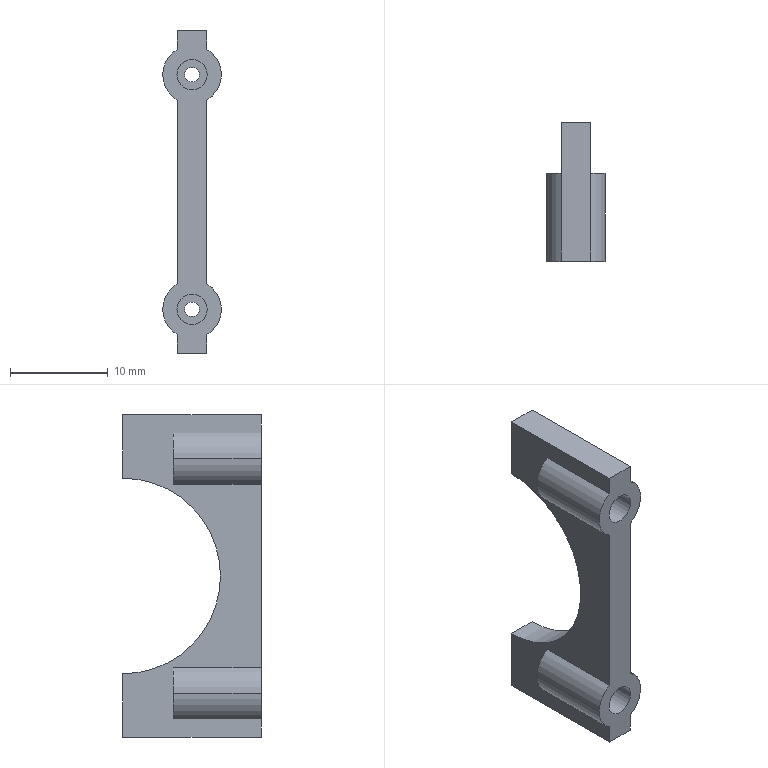Component | SolidWorks | Part10-2 | 1 solid | 29 faces | box 6 x 14.18 x 33 mm | volume 983 mm3 | cylinder 16 | plane 13 | commonest cylinder face diameters 6 x6 3.1 x4 1.5 x4 20 x2 | material 45
build123d program:
from build123d import *

# Parameters (mm, degrees)
BOSS_EXTRUDE1_DEPTH             = 3
SKETCH3_R                       = 0.75
CUT_EXTRUDE1_DEPTH              = 31.209
SKETCH1_R                       = 3
SKETCH1_R_2                     = 0.75
THREADBOSS_CHEESESCREW_DEPTH    = 9
SKETCH2_R                       = 1.55
TAPPEDHOLE_M3_CHEESESCREW_DEPTH = 8.5


with BuildPart() as part:
    # Sketch2_2 → Boss-Extrude1 (new body)
    with BuildSketch(Plane.XY):
        with BuildLine():
            Line((16.5, -26.504), (30.682, -26.504))
            Line((30.682, -26.504), (30.682, 6.496))
            Line((30.682, 6.496), (16.5, 6.496))
            Line((16.5, 6.496), (16.5, -0.004132))
            ThreePointArc((16.5, -0.004132), (26.5, -10.004), (16.5, -20.004))
            Line((16.5, -20.004), (16.5, -26.504))
        make_face()
    extrude(amount=-BOSS_EXTRUDE1_DEPTH)

    # Sketch3 → Cut-Extrude1 (cut, through all)
    with BuildSketch(Plane(origin=(30.682, 0, 0), x_dir=(0, 0, -1), z_dir=(1, 0, 0))):
        with Locations((1.5, -22.004)):
            Circle(SKETCH3_R)
        with Locations(Location((1.5, 1.996, 0), (0, 0, 180))):
            Circle(SKETCH3_R)
    extrude(amount=-CUT_EXTRUDE1_DEPTH, mode=Mode.SUBTRACT)

    # Sketch1 → ThreadBoss-CheeseScrew (add)
    # profile 1 of 2: a face of its own
    with BuildSketch(Plane(origin=(30.682, 0, 0), x_dir=(0, 0, -1), z_dir=(1, 0, 0))):
        with Locations((1.5, -22.004)):
            Circle(SKETCH1_R)
        with Locations((1.5, -22.004)):
            Circle(SKETCH1_R_2, mode=Mode.SUBTRACT)
    # profile 2 of 2: a face of its own
    with BuildSketch(Plane(origin=(30.682, 0, 0), x_dir=(0, 0, -1), z_dir=(1, 0, 0))):
        with Locations((1.5, 1.996)):
            Circle(SKETCH1_R)
        with Locations(Location((1.5, 1.996, 0), (0, 0, 180))):
            Circle(SKETCH1_R_2, mode=Mode.SUBTRACT)
    extrude(amount=-THREADBOSS_CHEESESCREW_DEPTH)

    # Sketch2 → TappedHole-M3-CheeseScrew (cut)
    with BuildSketch(Plane(origin=(30.682, 0, 0), x_dir=(0, 0, -1), z_dir=(1, 0, 0))):
        with Locations((1.5, -22.004)):
            Circle(SKETCH2_R)
        with Locations((1.5, 1.996)):
            Circle(SKETCH2_R)
    extrude(amount=-TAPPEDHOLE_M3_CHEESESCREW_DEPTH, mode=Mode.SUBTRACT)


solid = part.part

# Placed as in the assembly
solid = solid.moved(Location((-8.904, -28.5, 20.008), (90, -90, 0)))
STEP:
#1=COLOUR_RGB('',0.7922,0.8196,0.9333);
#2=FILL_AREA_STYLE_COLOUR('',#1);
#3=FILL_AREA_STYLE('',(#2));
#4=SURFACE_STYLE_FILL_AREA(#3);
#5=SURFACE_SIDE_STYLE('',(#4));
#6=SURFACE_STYLE_USAGE(.BOTH.,#5);
#7=PRESENTATION_STYLE_ASSIGNMENT((#6));
#8=CARTESIAN_POINT('',(-0.2305,-1.995,0.8663));
#9=VERTEX_POINT('',#8);
#10=CARTESIAN_POINT('',(-0.3525,-1.995,0.8663));
#11=VERTEX_POINT('',#10);
#12=CARTESIAN_POINT('',(-0.2915,-1.995,0.8663));
#13=DIRECTION('',(0.,-1.,0.));
#14=DIRECTION('',(-1.,0.,0.));
#15=AXIS2_PLACEMENT_3D('',#12,#13,#14);
#16=CIRCLE('',#15,0.06102);
#17=EDGE_CURVE('',#9,#11,#16,.T.);
#18=ORIENTED_EDGE('',*,*,#17,.F.);
#19=CARTESIAN_POINT('',(-0.2305,-2.33,0.8663));
#20=VERTEX_POINT('',#19);
#21=CARTESIAN_POINT('',(-0.2305,-1.995,0.8663));
#22=DIRECTION('',(0.,-1.,0.));
#23=VECTOR('',#22,39.37);
#24=LINE('',#21,#23);
#25=EDGE_CURVE('',#9,#20,#24,.T.);
#26=ORIENTED_EDGE('',*,*,#25,.T.);
#27=CARTESIAN_POINT('',(-0.3525,-2.33,0.8663));
#28=VERTEX_POINT('',#27);
#29=CARTESIAN_POINT('',(-0.2915,-2.33,0.8663));
#30=DIRECTION('',(0.,-1.,0.));
#31=DIRECTION('',(-1.,0.,0.));
#32=AXIS2_PLACEMENT_3D('',#29,#30,#31);
#33=CIRCLE('',#32,0.06102);
#34=EDGE_CURVE('',#20,#28,#33,.T.);
#35=ORIENTED_EDGE('',*,*,#34,.T.);
#36=CARTESIAN_POINT('',(-0.3525,-1.995,0.8663));
#37=DIRECTION('',(0.,-1.,0.));
#38=VECTOR('',#37,39.37);
#39=LINE('',#36,#38);
#40=EDGE_CURVE('',#11,#28,#39,.T.);
#41=ORIENTED_EDGE('',*,*,#40,.F.);
#42=EDGE_LOOP('',(#18,#26,#35,#41));
#43=FACE_OUTER_BOUND('',#42,.T.);
#44=CARTESIAN_POINT('',(-0.2915,-1.995,0.8663));
#45=DIRECTION('',(0.,-1.,0.));
#46=DIRECTION('',(-1.,0.,0.));
#47=AXIS2_PLACEMENT_3D('',#44,#45,#46);
#48=CYLINDRICAL_SURFACE('',#47,0.06102);
#49=ADVANCED_FACE('',(#43),#48,.F.);
#50=CARTESIAN_POINT('',(-0.2305,-1.995,-0.07858));
#51=VERTEX_POINT('',#50);
#52=CARTESIAN_POINT('',(-0.3525,-1.995,-0.07858));
#53=VERTEX_POINT('',#52);
#54=CARTESIAN_POINT('',(-0.2915,-1.995,-0.07858));
#55=DIRECTION('',(0.,-1.,0.));
#56=DIRECTION('',(-1.,0.,0.));
#57=AXIS2_PLACEMENT_3D('',#54,#55,#56);
#58=CIRCLE('',#57,0.06102);
#59=EDGE_CURVE('',#51,#53,#58,.T.);
#60=ORIENTED_EDGE('',*,*,#59,.F.);
#61=CARTESIAN_POINT('',(-0.2305,-2.33,-0.07858));
#62=VERTEX_POINT('',#61);
#63=CARTESIAN_POINT('',(-0.2305,-1.995,-0.07858));
#64=DIRECTION('',(0.,-1.,0.));
#65=VECTOR('',#64,39.37);
#66=LINE('',#63,#65);
#67=EDGE_CURVE('',#51,#62,#66,.T.);
#68=ORIENTED_EDGE('',*,*,#67,.T.);
#69=CARTESIAN_POINT('',(-0.3525,-2.33,-0.07858));
#70=VERTEX_POINT('',#69);
#71=CARTESIAN_POINT('',(-0.2915,-2.33,-0.07858));
#72=DIRECTION('',(0.,-1.,0.));
#73=DIRECTION('',(-1.,0.,0.));
#74=AXIS2_PLACEMENT_3D('',#71,#72,#73);
#75=CIRCLE('',#74,0.06102);
#76=EDGE_CURVE('',#62,#70,#75,.T.);
#77=ORIENTED_EDGE('',*,*,#76,.T.);
#78=CARTESIAN_POINT('',(-0.3525,-1.995,-0.07858));
#79=DIRECTION('',(0.,-1.,0.));
#80=VECTOR('',#79,39.37);
#81=LINE('',#78,#80);
#82=EDGE_CURVE('',#53,#70,#81,.T.);
#83=ORIENTED_EDGE('',*,*,#82,.F.);
#84=EDGE_LOOP('',(#60,#68,#77,#83));
#85=FACE_OUTER_BOUND('',#84,.T.);
#86=CARTESIAN_POINT('',(-0.2915,-1.995,-0.07858));
#87=DIRECTION('',(0.,-1.,0.));
#88=DIRECTION('',(-1.,0.,0.));
#89=AXIS2_PLACEMENT_3D('',#86,#87,#88);
#90=CYLINDRICAL_SURFACE('',#89,0.06102);
#91=ADVANCED_FACE('',(#85),#90,.F.);
#92=CARTESIAN_POINT('',(-0.3506,-1.976,0.9686));
#93=VERTEX_POINT('',#92);
#94=CARTESIAN_POINT('',(-0.4096,-1.976,0.8663));
#95=VERTEX_POINT('',#94);
#96=CARTESIAN_POINT('',(-0.2915,-1.976,0.8663));
#97=DIRECTION('',(0.,-1.,0.));
#98=DIRECTION('',(-1.,0.,0.));
#99=AXIS2_PLACEMENT_3D('',#96,#97,#98);
#100=CIRCLE('',#99,0.1181);
#101=EDGE_CURVE('',#93,#95,#100,.T.);
#102=ORIENTED_EDGE('',*,*,#101,.T.);
#103=CARTESIAN_POINT('',(-0.4096,-2.33,0.8663));
#104=VERTEX_POINT('',#103);
#105=CARTESIAN_POINT('',(-0.4096,-1.976,0.8663));
#106=DIRECTION('',(0.,-1.,0.));
#107=VECTOR('',#106,39.37);
#108=LINE('',#105,#107);
#109=EDGE_CURVE('',#95,#104,#108,.T.);
#110=ORIENTED_EDGE('',*,*,#109,.T.);
#111=CARTESIAN_POINT('',(-0.3506,-2.33,0.9686));
#112=VERTEX_POINT('',#111);
#113=CARTESIAN_POINT('',(-0.2915,-2.33,0.8663));
#114=DIRECTION('',(0.,-1.,0.));
#115=DIRECTION('',(-1.,0.,0.));
#116=AXIS2_PLACEMENT_3D('',#113,#114,#115);
#117=CIRCLE('',#116,0.1181);
#118=EDGE_CURVE('',#112,#104,#117,.T.);
#119=ORIENTED_EDGE('',*,*,#118,.F.);
#120=CARTESIAN_POINT('',(-0.3506,-1.976,0.9686));
#121=DIRECTION('',(0.,-1.,0.));
#122=VECTOR('',#121,39.37);
#123=LINE('',#120,#122);
#124=EDGE_CURVE('',#93,#112,#123,.T.);
#125=ORIENTED_EDGE('',*,*,#124,.F.);
#126=EDGE_LOOP('',(#102,#110,#119,#125));
#127=FACE_OUTER_BOUND('',#126,.T.);
#128=CARTESIAN_POINT('',(-0.2915,-1.976,0.8663));
#129=DIRECTION('',(0.,-1.,0.));
#130=DIRECTION('',(-1.,0.,0.));
#131=AXIS2_PLACEMENT_3D('',#128,#129,#130);
#132=CYLINDRICAL_SURFACE('',#131,0.1181);
#133=ADVANCED_FACE('',(#127),#132,.T.);
#134=CARTESIAN_POINT('',(-0.3506,-1.976,0.02371));
#135=VERTEX_POINT('',#134);
#136=CARTESIAN_POINT('',(-0.4096,-1.976,-0.07858));
#137=VERTEX_POINT('',#136);
#138=CARTESIAN_POINT('',(-0.2915,-1.976,-0.07858));
#139=DIRECTION('',(0.,-1.,0.));
#140=DIRECTION('',(-1.,0.,0.));
#141=AXIS2_PLACEMENT_3D('',#138,#139,#140);
#142=CIRCLE('',#141,0.1181);
#143=EDGE_CURVE('',#135,#137,#142,.T.);
#144=ORIENTED_EDGE('',*,*,#143,.T.);
#145=CARTESIAN_POINT('',(-0.4096,-2.33,-0.07858));
#146=VERTEX_POINT('',#145);
#147=CARTESIAN_POINT('',(-0.4096,-1.976,-0.07858));
#148=DIRECTION('',(0.,-1.,0.));
#149=VECTOR('',#148,39.37);
#150=LINE('',#147,#149);
#151=EDGE_CURVE('',#137,#146,#150,.T.);
#152=ORIENTED_EDGE('',*,*,#151,.T.);
#153=CARTESIAN_POINT('',(-0.3506,-2.33,0.02371));
#154=VERTEX_POINT('',#153);
#155=CARTESIAN_POINT('',(-0.2915,-2.33,-0.07858));
#156=DIRECTION('',(0.,-1.,0.));
#157=DIRECTION('',(-1.,0.,0.));
#158=AXIS2_PLACEMENT_3D('',#155,#156,#157);
#159=CIRCLE('',#158,0.1181);
#160=EDGE_CURVE('',#154,#146,#159,.T.);
#161=ORIENTED_EDGE('',*,*,#160,.F.);
#162=CARTESIAN_POINT('',(-0.3506,-1.976,0.02371));
#163=DIRECTION('',(0.,-1.,0.));
#164=VECTOR('',#163,39.37);
#165=LINE('',#162,#164);
#166=EDGE_CURVE('',#135,#154,#165,.T.);
#167=ORIENTED_EDGE('',*,*,#166,.F.);
#168=EDGE_LOOP('',(#144,#152,#161,#167));
#169=FACE_OUTER_BOUND('',#168,.T.);
#170=CARTESIAN_POINT('',(-0.2915,-1.976,-0.07858));
#171=DIRECTION('',(0.,-1.,0.));
#172=DIRECTION('',(-1.,0.,0.));
#173=AXIS2_PLACEMENT_3D('',#170,#171,#172);
#174=CYLINDRICAL_SURFACE('',#173,0.1181);
#175=ADVANCED_FACE('',(#169),#174,.T.);
#176=CARTESIAN_POINT('',(-0.3506,-1.772,0.0001627));
#177=VERTEX_POINT('',#176);
#178=CARTESIAN_POINT('',(-0.3506,-2.165,0.3939));
#179=VERTEX_POINT('',#178);
#180=CARTESIAN_POINT('',(-0.3506,-1.772,0.3939));
#181=DIRECTION('',(-1.,0.,0.));
#182=DIRECTION('',(0.,-1.,0.));
#183=AXIS2_PLACEMENT_3D('',#180,#181,#182);
#184=CIRCLE('',#183,0.3937);
#185=EDGE_CURVE('',#177,#179,#184,.T.);
#186=ORIENTED_EDGE('',*,*,#185,.T.);
#187=CARTESIAN_POINT('',(-0.2325,-2.165,0.3939));
#188=VERTEX_POINT('',#187);
#189=CARTESIAN_POINT('',(-0.3506,-2.165,0.3939));
#190=DIRECTION('',(1.,0.,0.));
#191=VECTOR('',#190,39.37);
#192=LINE('',#189,#191);
#193=EDGE_CURVE('',#179,#188,#192,.T.);
#194=ORIENTED_EDGE('',*,*,#193,.T.);
#195=CARTESIAN_POINT('',(-0.2325,-1.772,0.0001627));
#196=VERTEX_POINT('',#195);
#197=CARTESIAN_POINT('',(-0.2325,-1.772,0.3939));
#198=DIRECTION('',(-1.,0.,0.));
#199=DIRECTION('',(0.,-1.,0.));
#200=AXIS2_PLACEMENT_3D('',#197,#198,#199);
#201=CIRCLE('',#200,0.3937);
#202=EDGE_CURVE('',#196,#188,#201,.T.);
#203=ORIENTED_EDGE('',*,*,#202,.F.);
#204=CARTESIAN_POINT('',(-0.3506,-1.772,0.0001627));
#205=DIRECTION('',(1.,0.,0.));
#206=VECTOR('',#205,39.37);
#207=LINE('',#204,#206);
#208=EDGE_CURVE('',#177,#196,#207,.T.);
#209=ORIENTED_EDGE('',*,*,#208,.F.);
#210=EDGE_LOOP('',(#186,#194,#203,#209));
#211=FACE_OUTER_BOUND('',#210,.T.);
#212=CARTESIAN_POINT('',(-0.3506,-1.772,0.3939));
#213=DIRECTION('',(1.,0.,0.));
#214=DIRECTION('',(0.,-1.,0.));
#215=AXIS2_PLACEMENT_3D('',#212,#213,#214);
#216=CYLINDRICAL_SURFACE('',#215,0.3937);
#217=ADVANCED_FACE('',(#211),#216,.F.);
#218=CARTESIAN_POINT('',(-0.262,-1.772,-0.07858));
#219=VERTEX_POINT('',#218);
#220=CARTESIAN_POINT('',(-0.321,-1.772,-0.07858));
#221=VERTEX_POINT('',#220);
#222=CARTESIAN_POINT('',(-0.2915,-1.772,-0.07858));
#223=DIRECTION('',(0.,-1.,0.));
#224=DIRECTION('',(1.,0.,0.));
#225=AXIS2_PLACEMENT_3D('',#222,#223,#224);
#226=CIRCLE('',#225,0.02953);
#227=EDGE_CURVE('',#219,#221,#226,.T.);
#228=ORIENTED_EDGE('',*,*,#227,.F.);
#229=CARTESIAN_POINT('',(-0.262,-1.995,-0.07858));
#230=VERTEX_POINT('',#229);
#231=CARTESIAN_POINT('',(-0.262,-1.772,-0.07858));
#232=DIRECTION('',(0.,-1.,0.));
#233=VECTOR('',#232,39.37);
#234=LINE('',#231,#233);
#235=EDGE_CURVE('',#219,#230,#234,.T.);
#236=ORIENTED_EDGE('',*,*,#235,.T.);
#237=CARTESIAN_POINT('',(-0.321,-1.995,-0.07858));
#238=VERTEX_POINT('',#237);
#239=CARTESIAN_POINT('',(-0.2915,-1.995,-0.07858));
#240=DIRECTION('',(0.,1.,0.));
#241=DIRECTION('',(-1.,0.,0.));
#242=AXIS2_PLACEMENT_3D('',#239,#240,#241);
#243=CIRCLE('',#242,0.02953);
#244=EDGE_CURVE('',#238,#230,#243,.T.);
#245=ORIENTED_EDGE('',*,*,#244,.F.);
#246=CARTESIAN_POINT('',(-0.321,-1.772,-0.07858));
#247=DIRECTION('',(0.,-1.,0.));
#248=VECTOR('',#247,39.37);
#249=LINE('',#246,#248);
#250=EDGE_CURVE('',#221,#238,#249,.T.);
#251=ORIENTED_EDGE('',*,*,#250,.F.);
#252=EDGE_LOOP('',(#228,#236,#245,#251));
#253=FACE_OUTER_BOUND('',#252,.T.);
#254=CARTESIAN_POINT('',(-0.2915,-1.772,-0.07858));
#255=DIRECTION('',(0.,-1.,0.));
#256=DIRECTION('',(-1.,0.,0.));
#257=AXIS2_PLACEMENT_3D('',#254,#255,#256);
#258=CYLINDRICAL_SURFACE('',#257,0.02953);
#259=ADVANCED_FACE('',(#253),#258,.F.);
#260=CARTESIAN_POINT('',(-0.262,-1.772,0.8663));
#261=VERTEX_POINT('',#260);
#262=CARTESIAN_POINT('',(-0.321,-1.772,0.8663));
#263=VERTEX_POINT('',#262);
#264=CARTESIAN_POINT('',(-0.2915,-1.772,0.8663));
#265=DIRECTION('',(0.,-1.,0.));
#266=DIRECTION('',(-1.,0.,0.));
#267=AXIS2_PLACEMENT_3D('',#264,#265,#266);
#268=CIRCLE('',#267,0.02953);
#269=EDGE_CURVE('',#261,#263,#268,.T.);
#270=ORIENTED_EDGE('',*,*,#269,.F.);
#271=CARTESIAN_POINT('',(-0.262,-1.995,0.8663));
#272=VERTEX_POINT('',#271);
#273=CARTESIAN_POINT('',(-0.262,-1.772,0.8663));
#274=DIRECTION('',(0.,-1.,0.));
#275=VECTOR('',#274,39.37);
#276=LINE('',#273,#275);
#277=EDGE_CURVE('',#261,#272,#276,.T.);
#278=ORIENTED_EDGE('',*,*,#277,.T.);
#279=CARTESIAN_POINT('',(-0.321,-1.995,0.8663));
#280=VERTEX_POINT('',#279);
#281=CARTESIAN_POINT('',(-0.2915,-1.995,0.8663));
#282=DIRECTION('',(0.,1.,0.));
#283=DIRECTION('',(-1.,0.,0.));
#284=AXIS2_PLACEMENT_3D('',#281,#282,#283);
#285=CIRCLE('',#284,0.02953);
#286=EDGE_CURVE('',#280,#272,#285,.T.);
#287=ORIENTED_EDGE('',*,*,#286,.F.);
#288=CARTESIAN_POINT('',(-0.321,-1.772,0.8663));
#289=DIRECTION('',(0.,-1.,0.));
#290=VECTOR('',#289,39.37);
#291=LINE('',#288,#290);
#292=EDGE_CURVE('',#263,#280,#291,.T.);
#293=ORIENTED_EDGE('',*,*,#292,.F.);
#294=EDGE_LOOP('',(#270,#278,#287,#293));
#295=FACE_OUTER_BOUND('',#294,.T.);
#296=CARTESIAN_POINT('',(-0.2915,-1.772,0.8663));
#297=DIRECTION('',(0.,-1.,0.));
#298=DIRECTION('',(-1.,0.,0.));
#299=AXIS2_PLACEMENT_3D('',#296,#297,#298);
#300=CYLINDRICAL_SURFACE('',#299,0.02953);
#301=ADVANCED_FACE('',(#295),#300,.F.);
#302=ORIENTED_EDGE('',*,*,#277,.F.);
#303=CARTESIAN_POINT('',(-0.2915,-1.772,0.8663));
#304=DIRECTION('',(0.,-1.,0.));
#305=DIRECTION('',(-1.,0.,0.));
#306=AXIS2_PLACEMENT_3D('',#303,#304,#305);
#307=CIRCLE('',#306,0.02953);
#308=EDGE_CURVE('',#263,#261,#307,.T.);
#309=ORIENTED_EDGE('',*,*,#308,.F.);
#310=ORIENTED_EDGE('',*,*,#292,.T.);
#311=CARTESIAN_POINT('',(-0.2915,-1.995,0.8663));
#312=DIRECTION('',(0.,1.,0.));
#313=DIRECTION('',(-1.,0.,0.));
#314=AXIS2_PLACEMENT_3D('',#311,#312,#313);
#315=CIRCLE('',#314,0.02953);
#316=EDGE_CURVE('',#272,#280,#315,.T.);
#317=ORIENTED_EDGE('',*,*,#316,.F.);
#318=EDGE_LOOP('',(#302,#309,#310,#317));
#319=FACE_OUTER_BOUND('',#318,.T.);
#320=CARTESIAN_POINT('',(-0.2915,-1.772,0.8663));
#321=DIRECTION('',(0.,-1.,0.));
#322=DIRECTION('',(-1.,0.,0.));
#323=AXIS2_PLACEMENT_3D('',#320,#321,#322);
#324=CYLINDRICAL_SURFACE('',#323,0.02953);
#325=ADVANCED_FACE('',(#319),#324,.F.);
#326=ORIENTED_EDGE('',*,*,#235,.F.);
#327=CARTESIAN_POINT('',(-0.2915,-1.772,-0.07858));
#328=DIRECTION('',(0.,-1.,0.));
#329=DIRECTION('',(1.,0.,0.));
#330=AXIS2_PLACEMENT_3D('',#327,#328,#329);
#331=CIRCLE('',#330,0.02953);
#332=EDGE_CURVE('',#221,#219,#331,.T.);
#333=ORIENTED_EDGE('',*,*,#332,.F.);
#334=ORIENTED_EDGE('',*,*,#250,.T.);
#335=CARTESIAN_POINT('',(-0.2915,-1.995,-0.07858));
#336=DIRECTION('',(0.,1.,0.));
#337=DIRECTION('',(-1.,0.,0.));
#338=AXIS2_PLACEMENT_3D('',#335,#336,#337);
#339=CIRCLE('',#338,0.02953);
#340=EDGE_CURVE('',#230,#238,#339,.T.);
#341=ORIENTED_EDGE('',*,*,#340,.F.);
#342=EDGE_LOOP('',(#326,#333,#334,#341));
#343=FACE_OUTER_BOUND('',#342,.T.);
#344=CARTESIAN_POINT('',(-0.2915,-1.772,-0.07858));
#345=DIRECTION('',(0.,-1.,0.));
#346=DIRECTION('',(-1.,0.,0.));
#347=AXIS2_PLACEMENT_3D('',#344,#345,#346);
#348=CYLINDRICAL_SURFACE('',#347,0.02953);
#349=ADVANCED_FACE('',(#343),#348,.F.);
#350=ORIENTED_EDGE('',*,*,#308,.T.);
#351=ORIENTED_EDGE('',*,*,#269,.T.);
#352=EDGE_LOOP('',(#350,#351));
#353=FACE_BOUND('',#352,.T.);
#354=CARTESIAN_POINT('',(-0.2325,-1.772,0.7876));
#355=VERTEX_POINT('',#354);
#356=CARTESIAN_POINT('',(-0.2325,-1.772,1.043));
#357=VERTEX_POINT('',#356);
#358=CARTESIAN_POINT('',(-0.2325,-1.772,1.043));
#359=DIRECTION('',(0.,0.,1.));
#360=VECTOR('',#359,39.37);
#361=LINE('',#358,#360);
#362=EDGE_CURVE('',#355,#357,#361,.T.);
#363=ORIENTED_EDGE('',*,*,#362,.F.);
#364=CARTESIAN_POINT('',(-0.3506,-1.772,0.7876));
#365=VERTEX_POINT('',#364);
#366=CARTESIAN_POINT('',(-0.3506,-1.772,0.7876));
#367=DIRECTION('',(1.,0.,0.));
#368=VECTOR('',#367,39.37);
#369=LINE('',#366,#368);
#370=EDGE_CURVE('',#365,#355,#369,.T.);
#371=ORIENTED_EDGE('',*,*,#370,.F.);
#372=CARTESIAN_POINT('',(-0.3506,-1.772,1.043));
#373=VERTEX_POINT('',#372);
#374=CARTESIAN_POINT('',(-0.3506,-1.772,1.043));
#375=DIRECTION('',(0.,0.,1.));
#376=VECTOR('',#375,39.37);
#377=LINE('',#374,#376);
#378=EDGE_CURVE('',#365,#373,#377,.T.);
#379=ORIENTED_EDGE('',*,*,#378,.T.);
#380=CARTESIAN_POINT('',(-0.3506,-1.772,1.043));
#381=DIRECTION('',(1.,0.,0.));
#382=VECTOR('',#381,39.37);
#383=LINE('',#380,#382);
#384=EDGE_CURVE('',#373,#357,#383,.T.);
#385=ORIENTED_EDGE('',*,*,#384,.T.);
#386=EDGE_LOOP('',(#363,#371,#379,#385));
#387=FACE_OUTER_BOUND('',#386,.T.);
#388=CARTESIAN_POINT('',(-0.3506,-1.772,1.043));
#389=DIRECTION('',(0.,1.,0.));
#390=DIRECTION('',(1.,0.,0.));
#391=AXIS2_PLACEMENT_3D('',#388,#389,#390);
#392=PLANE('',#391);
#393=ADVANCED_FACE('',(#353,#387),#392,.T.);
#394=ORIENTED_EDGE('',*,*,#193,.F.);
#395=CARTESIAN_POINT('',(-0.3506,-1.772,0.3939));
#396=DIRECTION('',(-1.,0.,0.));
#397=DIRECTION('',(0.,-1.,0.));
#398=AXIS2_PLACEMENT_3D('',#395,#396,#397);
#399=CIRCLE('',#398,0.3937);
#400=EDGE_CURVE('',#179,#365,#399,.T.);
#401=ORIENTED_EDGE('',*,*,#400,.T.);
#402=ORIENTED_EDGE('',*,*,#370,.T.);
#403=CARTESIAN_POINT('',(-0.2325,-1.772,0.3939));
#404=DIRECTION('',(-1.,0.,0.));
#405=DIRECTION('',(0.,-1.,0.));
#406=AXIS2_PLACEMENT_3D('',#403,#404,#405);
#407=CIRCLE('',#406,0.3937);
#408=EDGE_CURVE('',#188,#355,#407,.T.);
#409=ORIENTED_EDGE('',*,*,#408,.F.);
#410=EDGE_LOOP('',(#394,#401,#402,#409));
#411=FACE_OUTER_BOUND('',#410,.T.);
#412=CARTESIAN_POINT('',(-0.3506,-1.772,0.3939));
#413=DIRECTION('',(1.,0.,0.));
#414=DIRECTION('',(0.,-1.,0.));
#415=AXIS2_PLACEMENT_3D('',#412,#413,#414);
#416=CYLINDRICAL_SURFACE('',#415,0.3937);
#417=ADVANCED_FACE('',(#411),#416,.F.);
#418=ORIENTED_EDGE('',*,*,#332,.T.);
#419=ORIENTED_EDGE('',*,*,#227,.T.);
#420=EDGE_LOOP('',(#418,#419));
#421=FACE_BOUND('',#420,.T.);
#422=CARTESIAN_POINT('',(-0.2325,-1.772,-0.2557));
#423=VERTEX_POINT('',#422);
#424=CARTESIAN_POINT('',(-0.2325,-1.772,-0.2557));
#425=DIRECTION('',(0.,0.,1.));
#426=VECTOR('',#425,39.37);
#427=LINE('',#424,#426);
#428=EDGE_CURVE('',#423,#196,#427,.T.);
#429=ORIENTED_EDGE('',*,*,#428,.F.);
#430=CARTESIAN_POINT('',(-0.3506,-1.772,-0.2557));
#431=VERTEX_POINT('',#430);
#432=CARTESIAN_POINT('',(-0.3506,-1.772,-0.2557));
#433=DIRECTION('',(1.,0.,0.));
#434=VECTOR('',#433,39.37);
#435=LINE('',#432,#434);
#436=EDGE_CURVE('',#431,#423,#435,.T.);
#437=ORIENTED_EDGE('',*,*,#436,.F.);
#438=CARTESIAN_POINT('',(-0.3506,-1.772,-0.2557));
#439=DIRECTION('',(0.,0.,1.));
#440=VECTOR('',#439,39.37);
#441=LINE('',#438,#440);
#442=EDGE_CURVE('',#431,#177,#441,.T.);
#443=ORIENTED_EDGE('',*,*,#442,.T.);
#444=ORIENTED_EDGE('',*,*,#208,.T.);
#445=EDGE_LOOP('',(#429,#437,#443,#444));
#446=FACE_OUTER_BOUND('',#445,.T.);
#447=CARTESIAN_POINT('',(-0.3506,-1.772,-0.2557));
#448=DIRECTION('',(0.,1.,0.));
#449=DIRECTION('',(1.,0.,0.));
#450=AXIS2_PLACEMENT_3D('',#447,#448,#449);
#451=PLANE('',#450);
#452=ADVANCED_FACE('',(#421,#446),#451,.T.);
#453=CARTESIAN_POINT('',(-0.2325,-2.33,-0.2557));
#454=VERTEX_POINT('',#453);
#455=CARTESIAN_POINT('',(-0.2325,-2.33,-0.2557));
#456=DIRECTION('',(0.,1.,0.));
#457=VECTOR('',#456,39.37);
#458=LINE('',#455,#457);
#459=EDGE_CURVE('',#454,#423,#458,.T.);
#460=ORIENTED_EDGE('',*,*,#459,.F.);
#461=CARTESIAN_POINT('',(-0.3506,-2.33,-0.2557));
#462=VERTEX_POINT('',#461);
#463=CARTESIAN_POINT('',(-0.3506,-2.33,-0.2557));
#464=DIRECTION('',(1.,0.,0.));
#465=VECTOR('',#464,39.37);
#466=LINE('',#463,#465);
#467=EDGE_CURVE('',#462,#454,#466,.T.);
#468=ORIENTED_EDGE('',*,*,#467,.F.);
#469=CARTESIAN_POINT('',(-0.3506,-2.33,-0.2557));
#470=DIRECTION('',(0.,1.,0.));
#471=VECTOR('',#470,39.37);
#472=LINE('',#469,#471);
#473=EDGE_CURVE('',#462,#431,#472,.T.);
#474=ORIENTED_EDGE('',*,*,#473,.T.);
#475=ORIENTED_EDGE('',*,*,#436,.T.);
#476=EDGE_LOOP('',(#460,#468,#474,#475));
#477=FACE_OUTER_BOUND('',#476,.T.);
#478=CARTESIAN_POINT('',(-0.3506,-2.33,-0.2557));
#479=DIRECTION('',(0.,0.,-1.));
#480=DIRECTION('',(1.,0.,0.));
#481=AXIS2_PLACEMENT_3D('',#478,#479,#480);
#482=PLANE('',#481);
#483=ADVANCED_FACE('',(#477),#482,.T.);
#484=CARTESIAN_POINT('',(-0.2915,-2.33,0.8663));
#485=DIRECTION('',(0.,-1.,0.));
#486=DIRECTION('',(-1.,0.,0.));
#487=AXIS2_PLACEMENT_3D('',#484,#485,#486);
#488=CIRCLE('',#487,0.06102);
#489=EDGE_CURVE('',#28,#20,#488,.T.);
#490=ORIENTED_EDGE('',*,*,#489,.F.);
#491=ORIENTED_EDGE('',*,*,#34,.F.);
#492=EDGE_LOOP('',(#490,#491));
#493=FACE_BOUND('',#492,.T.);
#494=CARTESIAN_POINT('',(-0.2915,-2.33,-0.07858));
#495=DIRECTION('',(0.,-1.,0.));
#496=DIRECTION('',(-1.,0.,0.));
#497=AXIS2_PLACEMENT_3D('',#494,#495,#496);
#498=CIRCLE('',#497,0.06102);
#499=EDGE_CURVE('',#70,#62,#498,.T.);
#500=ORIENTED_EDGE('',*,*,#499,.F.);
#501=ORIENTED_EDGE('',*,*,#76,.F.);
#502=EDGE_LOOP('',(#500,#501));
#503=FACE_BOUND('',#502,.T.);
#504=CARTESIAN_POINT('',(-0.3506,-2.33,1.043));
#505=VERTEX_POINT('',#504);
#506=CARTESIAN_POINT('',(-0.3506,-2.33,1.043));
#507=DIRECTION('',(0.,0.,-1.));
#508=VECTOR('',#507,39.37);
#509=LINE('',#506,#508);
#510=EDGE_CURVE('',#505,#112,#509,.T.);
#511=ORIENTED_EDGE('',*,*,#510,.T.);
#512=ORIENTED_EDGE('',*,*,#118,.T.);
#513=CARTESIAN_POINT('',(-0.3506,-2.33,0.764));
#514=VERTEX_POINT('',#513);
#515=CARTESIAN_POINT('',(-0.2915,-2.33,0.8663));
#516=DIRECTION('',(0.,-1.,0.));
#517=DIRECTION('',(-1.,0.,0.));
#518=AXIS2_PLACEMENT_3D('',#515,#516,#517);
#519=CIRCLE('',#518,0.1181);
#520=EDGE_CURVE('',#104,#514,#519,.T.);
#521=ORIENTED_EDGE('',*,*,#520,.T.);
#522=CARTESIAN_POINT('',(-0.3506,-2.33,1.043));
#523=DIRECTION('',(0.,0.,-1.));
#524=VECTOR('',#523,39.37);
#525=LINE('',#522,#524);
#526=EDGE_CURVE('',#514,#154,#525,.T.);
#527=ORIENTED_EDGE('',*,*,#526,.T.);
#528=ORIENTED_EDGE('',*,*,#160,.T.);
#529=CARTESIAN_POINT('',(-0.3506,-2.33,-0.1809));
#530=VERTEX_POINT('',#529);
#531=CARTESIAN_POINT('',(-0.2915,-2.33,-0.07858));
#532=DIRECTION('',(0.,-1.,0.));
#533=DIRECTION('',(-1.,0.,0.));
#534=AXIS2_PLACEMENT_3D('',#531,#532,#533);
#535=CIRCLE('',#534,0.1181);
#536=EDGE_CURVE('',#146,#530,#535,.T.);
#537=ORIENTED_EDGE('',*,*,#536,.T.);
#538=CARTESIAN_POINT('',(-0.3506,-2.33,1.043));
#539=DIRECTION('',(0.,0.,-1.));
#540=VECTOR('',#539,39.37);
#541=LINE('',#538,#540);
#542=EDGE_CURVE('',#530,#462,#541,.T.);
#543=ORIENTED_EDGE('',*,*,#542,.T.);
#544=ORIENTED_EDGE('',*,*,#467,.T.);
#545=CARTESIAN_POINT('',(-0.2325,-2.33,-0.1809));
#546=VERTEX_POINT('',#545);
#547=CARTESIAN_POINT('',(-0.2325,-2.33,1.043));
#548=DIRECTION('',(0.,0.,-1.));
#549=VECTOR('',#548,39.37);
#550=LINE('',#547,#549);
#551=EDGE_CURVE('',#546,#454,#550,.T.);
#552=ORIENTED_EDGE('',*,*,#551,.F.);
#553=CARTESIAN_POINT('',(-0.2325,-2.33,0.02371));
#554=VERTEX_POINT('',#553);
#555=CARTESIAN_POINT('',(-0.2915,-2.33,-0.07858));
#556=DIRECTION('',(0.,-1.,0.));
#557=DIRECTION('',(-1.,0.,0.));
#558=AXIS2_PLACEMENT_3D('',#555,#556,#557);
#559=CIRCLE('',#558,0.1181);
#560=EDGE_CURVE('',#546,#554,#559,.T.);
#561=ORIENTED_EDGE('',*,*,#560,.T.);
#562=CARTESIAN_POINT('',(-0.2325,-2.33,0.764));
#563=VERTEX_POINT('',#562);
#564=CARTESIAN_POINT('',(-0.2325,-2.33,1.043));
#565=DIRECTION('',(0.,0.,-1.));
#566=VECTOR('',#565,39.37);
#567=LINE('',#564,#566);
#568=EDGE_CURVE('',#563,#554,#567,.T.);
#569=ORIENTED_EDGE('',*,*,#568,.F.);
#570=CARTESIAN_POINT('',(-0.2325,-2.33,0.9686));
#571=VERTEX_POINT('',#570);
#572=CARTESIAN_POINT('',(-0.2915,-2.33,0.8663));
#573=DIRECTION('',(0.,-1.,0.));
#574=DIRECTION('',(-1.,0.,0.));
#575=AXIS2_PLACEMENT_3D('',#572,#573,#574);
#576=CIRCLE('',#575,0.1181);
#577=EDGE_CURVE('',#563,#571,#576,.T.);
#578=ORIENTED_EDGE('',*,*,#577,.T.);
#579=CARTESIAN_POINT('',(-0.2325,-2.33,1.043));
#580=VERTEX_POINT('',#579);
#581=CARTESIAN_POINT('',(-0.2325,-2.33,1.043));
#582=DIRECTION('',(0.,0.,-1.));
#583=VECTOR('',#582,39.37);
#584=LINE('',#581,#583);
#585=EDGE_CURVE('',#580,#571,#584,.T.);
#586=ORIENTED_EDGE('',*,*,#585,.F.);
#587=CARTESIAN_POINT('',(-0.3506,-2.33,1.043));
#588=DIRECTION('',(1.,0.,0.));
#589=VECTOR('',#588,39.37);
#590=LINE('',#587,#589);
#591=EDGE_CURVE('',#505,#580,#590,.T.);
#592=ORIENTED_EDGE('',*,*,#591,.F.);
#593=EDGE_LOOP('',(#511,#512,#521,#527,#528,#537,#543,#544,#552,#561,#569,#578,#586,#592));
#594=FACE_OUTER_BOUND('',#593,.T.);
#595=CARTESIAN_POINT('',(-0.3506,-2.33,1.043));
#596=DIRECTION('',(0.,-1.,0.));
#597=DIRECTION('',(-1.,0.,0.));
#598=AXIS2_PLACEMENT_3D('',#595,#596,#597);
#599=PLANE('',#598);
#600=ADVANCED_FACE('',(#493,#503,#594),#599,.T.);
#601=CARTESIAN_POINT('',(-0.2325,-1.772,1.043));
#602=DIRECTION('',(0.,-1.,0.));
#603=VECTOR('',#602,39.37);
#604=LINE('',#601,#603);
#605=EDGE_CURVE('',#357,#580,#604,.T.);
#606=ORIENTED_EDGE('',*,*,#605,.F.);
#607=ORIENTED_EDGE('',*,*,#384,.F.);
#608=CARTESIAN_POINT('',(-0.3506,-1.772,1.043));
#609=DIRECTION('',(0.,-1.,0.));
#610=VECTOR('',#609,39.37);
#611=LINE('',#608,#610);
#612=EDGE_CURVE('',#373,#505,#611,.T.);
#613=ORIENTED_EDGE('',*,*,#612,.T.);
#614=ORIENTED_EDGE('',*,*,#591,.T.);
#615=EDGE_LOOP('',(#606,#607,#613,#614));
#616=FACE_OUTER_BOUND('',#615,.T.);
#617=CARTESIAN_POINT('',(-0.3506,-1.772,1.043));
#618=DIRECTION('',(0.,0.,1.));
#619=DIRECTION('',(-1.,0.,0.));
#620=AXIS2_PLACEMENT_3D('',#617,#618,#619);
#621=PLANE('',#620);
#622=ADVANCED_FACE('',(#616),#621,.T.);
#623=CARTESIAN_POINT('',(-0.3506,-1.976,0.764));
#624=VERTEX_POINT('',#623);
#625=CARTESIAN_POINT('',(-0.3506,-1.976,0.3939));
#626=DIRECTION('',(0.,0.,-1.));
#627=VECTOR('',#626,39.37);
#628=LINE('',#625,#627);
#629=EDGE_CURVE('',#93,#624,#628,.T.);
#630=ORIENTED_EDGE('',*,*,#629,.F.);
#631=ORIENTED_EDGE('',*,*,#124,.T.);
#632=ORIENTED_EDGE('',*,*,#510,.F.);
#633=ORIENTED_EDGE('',*,*,#612,.F.);
#634=ORIENTED_EDGE('',*,*,#378,.F.);
#635=ORIENTED_EDGE('',*,*,#400,.F.);
#636=ORIENTED_EDGE('',*,*,#185,.F.);
#637=ORIENTED_EDGE('',*,*,#442,.F.);
#638=ORIENTED_EDGE('',*,*,#473,.F.);
#639=ORIENTED_EDGE('',*,*,#542,.F.);
#640=CARTESIAN_POINT('',(-0.3506,-1.976,-0.1809));
#641=VERTEX_POINT('',#640);
#642=CARTESIAN_POINT('',(-0.3506,-1.976,-0.1809));
#643=DIRECTION('',(0.,1.,0.));
#644=VECTOR('',#643,39.37);
#645=LINE('',#642,#644);
#646=EDGE_CURVE('',#530,#641,#645,.T.);
#647=ORIENTED_EDGE('',*,*,#646,.T.);
#648=CARTESIAN_POINT('',(-0.3506,-1.976,0.3939));
#649=DIRECTION('',(0.,0.,-1.));
#650=VECTOR('',#649,39.37);
#651=LINE('',#648,#650);
#652=EDGE_CURVE('',#135,#641,#651,.T.);
#653=ORIENTED_EDGE('',*,*,#652,.F.);
#654=ORIENTED_EDGE('',*,*,#166,.T.);
#655=ORIENTED_EDGE('',*,*,#526,.F.);
#656=CARTESIAN_POINT('',(-0.3506,-1.976,0.764));
#657=DIRECTION('',(0.,1.,0.));
#658=VECTOR('',#657,39.37);
#659=LINE('',#656,#658);
#660=EDGE_CURVE('',#514,#624,#659,.T.);
#661=ORIENTED_EDGE('',*,*,#660,.T.);
#662=EDGE_LOOP('',(#630,#631,#632,#633,#634,#635,#636,#637,#638,#639,#647,#653,#654,#655,#661));
#663=FACE_OUTER_BOUND('',#662,.T.);
#664=CARTESIAN_POINT('',(-0.3506,-1.772,0.3939));
#665=DIRECTION('',(1.,0.,0.));
#666=DIRECTION('',(0.,-1.,0.));
#667=AXIS2_PLACEMENT_3D('',#664,#665,#666);
#668=PLANE('',#667);
#669=ADVANCED_FACE('',(#663),#668,.F.);
#670=CARTESIAN_POINT('',(-0.2325,-1.976,0.9686));
#671=VERTEX_POINT('',#670);
#672=CARTESIAN_POINT('',(-0.2325,-1.976,0.9686));
#673=DIRECTION('',(0.,-1.,0.));
#674=VECTOR('',#673,39.37);
#675=LINE('',#672,#674);
#676=EDGE_CURVE('',#671,#571,#675,.T.);
#677=ORIENTED_EDGE('',*,*,#676,.F.);
#678=CARTESIAN_POINT('',(-0.2325,-1.976,0.764));
#679=VERTEX_POINT('',#678);
#680=CARTESIAN_POINT('',(-0.2325,-1.976,0.3939));
#681=DIRECTION('',(0.,0.,-1.));
#682=VECTOR('',#681,39.37);
#683=LINE('',#680,#682);
#684=EDGE_CURVE('',#671,#679,#683,.T.);
#685=ORIENTED_EDGE('',*,*,#684,.T.);
#686=CARTESIAN_POINT('',(-0.2325,-1.976,0.764));
#687=DIRECTION('',(0.,1.,0.));
#688=VECTOR('',#687,39.37);
#689=LINE('',#686,#688);
#690=EDGE_CURVE('',#563,#679,#689,.T.);
#691=ORIENTED_EDGE('',*,*,#690,.F.);
#692=ORIENTED_EDGE('',*,*,#568,.T.);
#693=CARTESIAN_POINT('',(-0.2325,-1.976,0.02371));
#694=VERTEX_POINT('',#693);
#695=CARTESIAN_POINT('',(-0.2325,-1.976,0.02371));
#696=DIRECTION('',(0.,-1.,0.));
#697=VECTOR('',#696,39.37);
#698=LINE('',#695,#697);
#699=EDGE_CURVE('',#694,#554,#698,.T.);
#700=ORIENTED_EDGE('',*,*,#699,.F.);
#701=CARTESIAN_POINT('',(-0.2325,-1.976,-0.1809));
#702=VERTEX_POINT('',#701);
#703=CARTESIAN_POINT('',(-0.2325,-1.976,0.3939));
#704=DIRECTION('',(0.,0.,-1.));
#705=VECTOR('',#704,39.37);
#706=LINE('',#703,#705);
#707=EDGE_CURVE('',#694,#702,#706,.T.);
#708=ORIENTED_EDGE('',*,*,#707,.T.);
#709=CARTESIAN_POINT('',(-0.2325,-1.976,-0.1809));
#710=DIRECTION('',(0.,1.,0.));
#711=VECTOR('',#710,39.37);
#712=LINE('',#709,#711);
#713=EDGE_CURVE('',#546,#702,#712,.T.);
#714=ORIENTED_EDGE('',*,*,#713,.F.);
#715=ORIENTED_EDGE('',*,*,#551,.T.);
#716=ORIENTED_EDGE('',*,*,#459,.T.);
#717=ORIENTED_EDGE('',*,*,#428,.T.);
#718=ORIENTED_EDGE('',*,*,#202,.T.);
#719=ORIENTED_EDGE('',*,*,#408,.T.);
#720=ORIENTED_EDGE('',*,*,#362,.T.);
#721=ORIENTED_EDGE('',*,*,#605,.T.);
#722=ORIENTED_EDGE('',*,*,#585,.T.);
#723=EDGE_LOOP('',(#677,#685,#691,#692,#700,#708,#714,#715,#716,#717,#718,#719,#720,#721,#722));
#724=FACE_OUTER_BOUND('',#723,.T.);
#725=CARTESIAN_POINT('',(-0.2325,-1.772,0.3939));
#726=DIRECTION('',(1.,0.,0.));
#727=DIRECTION('',(0.,-1.,0.));
#728=AXIS2_PLACEMENT_3D('',#725,#726,#727);
#729=PLANE('',#728);
#730=ADVANCED_FACE('',(#724),#729,.T.);
#731=ORIENTED_EDGE('',*,*,#707,.F.);
#732=CARTESIAN_POINT('',(-0.2915,-1.976,-0.07858));
#733=DIRECTION('',(0.,-1.,0.));
#734=DIRECTION('',(-1.,0.,0.));
#735=AXIS2_PLACEMENT_3D('',#732,#733,#734);
#736=CIRCLE('',#735,0.1181);
#737=EDGE_CURVE('',#702,#694,#736,.T.);
#738=ORIENTED_EDGE('',*,*,#737,.F.);
#739=EDGE_LOOP('',(#731,#738));
#740=FACE_OUTER_BOUND('',#739,.T.);
#741=CARTESIAN_POINT('',(-0.2915,-1.976,-0.07858));
#742=DIRECTION('',(0.,-1.,0.));
#743=DIRECTION('',(-1.,0.,0.));
#744=AXIS2_PLACEMENT_3D('',#741,#742,#743);
#745=PLANE('',#744);
#746=ADVANCED_FACE('',(#740),#745,.F.);
#747=ORIENTED_EDGE('',*,*,#737,.T.);
#748=ORIENTED_EDGE('',*,*,#699,.T.);
#749=ORIENTED_EDGE('',*,*,#560,.F.);
#750=ORIENTED_EDGE('',*,*,#713,.T.);
#751=EDGE_LOOP('',(#747,#748,#749,#750));
#752=FACE_OUTER_BOUND('',#751,.T.);
#753=CARTESIAN_POINT('',(-0.2915,-1.976,-0.07858));
#754=DIRECTION('',(0.,-1.,0.));
#755=DIRECTION('',(-1.,0.,0.));
#756=AXIS2_PLACEMENT_3D('',#753,#754,#755);
#757=CYLINDRICAL_SURFACE('',#756,0.1181);
#758=ADVANCED_FACE('',(#752),#757,.T.);
#759=ORIENTED_EDGE('',*,*,#684,.F.);
#760=CARTESIAN_POINT('',(-0.2915,-1.976,0.8663));
#761=DIRECTION('',(0.,-1.,0.));
#762=DIRECTION('',(-1.,0.,0.));
#763=AXIS2_PLACEMENT_3D('',#760,#761,#762);
#764=CIRCLE('',#763,0.1181);
#765=EDGE_CURVE('',#679,#671,#764,.T.);
#766=ORIENTED_EDGE('',*,*,#765,.F.);
#767=EDGE_LOOP('',(#759,#766));
#768=FACE_OUTER_BOUND('',#767,.T.);
#769=CARTESIAN_POINT('',(-0.2915,-1.976,0.8663));
#770=DIRECTION('',(0.,-1.,0.));
#771=DIRECTION('',(-1.,0.,0.));
#772=AXIS2_PLACEMENT_3D('',#769,#770,#771);
#773=PLANE('',#772);
#774=ADVANCED_FACE('',(#768),#773,.F.);
#775=ORIENTED_EDGE('',*,*,#765,.T.);
#776=ORIENTED_EDGE('',*,*,#676,.T.);
#777=ORIENTED_EDGE('',*,*,#577,.F.);
#778=ORIENTED_EDGE('',*,*,#690,.T.);
#779=EDGE_LOOP('',(#775,#776,#777,#778));
#780=FACE_OUTER_BOUND('',#779,.T.);
#781=CARTESIAN_POINT('',(-0.2915,-1.976,0.8663));
#782=DIRECTION('',(0.,-1.,0.));
#783=DIRECTION('',(-1.,0.,0.));
#784=AXIS2_PLACEMENT_3D('',#781,#782,#783);
#785=CYLINDRICAL_SURFACE('',#784,0.1181);
#786=ADVANCED_FACE('',(#780),#785,.T.);
#787=ORIENTED_EDGE('',*,*,#151,.F.);
#788=CARTESIAN_POINT('',(-0.2915,-1.976,-0.07858));
#789=DIRECTION('',(0.,-1.,0.));
#790=DIRECTION('',(-1.,0.,0.));
#791=AXIS2_PLACEMENT_3D('',#788,#789,#790);
#792=CIRCLE('',#791,0.1181);
#793=EDGE_CURVE('',#137,#641,#792,.T.);
#794=ORIENTED_EDGE('',*,*,#793,.T.);
#795=ORIENTED_EDGE('',*,*,#646,.F.);
#796=ORIENTED_EDGE('',*,*,#536,.F.);
#797=EDGE_LOOP('',(#787,#794,#795,#796));
#798=FACE_OUTER_BOUND('',#797,.T.);
#799=CARTESIAN_POINT('',(-0.2915,-1.976,-0.07858));
#800=DIRECTION('',(0.,-1.,0.));
#801=DIRECTION('',(-1.,0.,0.));
#802=AXIS2_PLACEMENT_3D('',#799,#800,#801);
#803=CYLINDRICAL_SURFACE('',#802,0.1181);
#804=ADVANCED_FACE('',(#798),#803,.T.);
#805=ORIENTED_EDGE('',*,*,#143,.F.);
#806=ORIENTED_EDGE('',*,*,#652,.T.);
#807=ORIENTED_EDGE('',*,*,#793,.F.);
#808=EDGE_LOOP('',(#805,#806,#807));
#809=FACE_OUTER_BOUND('',#808,.T.);
#810=CARTESIAN_POINT('',(-0.2915,-1.976,-0.07858));
#811=DIRECTION('',(0.,-1.,0.));
#812=DIRECTION('',(-1.,0.,0.));
#813=AXIS2_PLACEMENT_3D('',#810,#811,#812);
#814=PLANE('',#813);
#815=ADVANCED_FACE('',(#809),#814,.F.);
#816=ORIENTED_EDGE('',*,*,#109,.F.);
#817=CARTESIAN_POINT('',(-0.2915,-1.976,0.8663));
#818=DIRECTION('',(0.,-1.,0.));
#819=DIRECTION('',(-1.,0.,0.));
#820=AXIS2_PLACEMENT_3D('',#817,#818,#819);
#821=CIRCLE('',#820,0.1181);
#822=EDGE_CURVE('',#95,#624,#821,.T.);
#823=ORIENTED_EDGE('',*,*,#822,.T.);
#824=ORIENTED_EDGE('',*,*,#660,.F.);
#825=ORIENTED_EDGE('',*,*,#520,.F.);
#826=EDGE_LOOP('',(#816,#823,#824,#825));
#827=FACE_OUTER_BOUND('',#826,.T.);
#828=CARTESIAN_POINT('',(-0.2915,-1.976,0.8663));
#829=DIRECTION('',(0.,-1.,0.));
#830=DIRECTION('',(-1.,0.,0.));
#831=AXIS2_PLACEMENT_3D('',#828,#829,#830);
#832=CYLINDRICAL_SURFACE('',#831,0.1181);
#833=ADVANCED_FACE('',(#827),#832,.T.);
#834=ORIENTED_EDGE('',*,*,#101,.F.);
#835=ORIENTED_EDGE('',*,*,#629,.T.);
#836=ORIENTED_EDGE('',*,*,#822,.F.);
#837=EDGE_LOOP('',(#834,#835,#836));
#838=FACE_OUTER_BOUND('',#837,.T.);
#839=CARTESIAN_POINT('',(-0.2915,-1.976,0.8663));
#840=DIRECTION('',(0.,-1.,0.));
#841=DIRECTION('',(-1.,0.,0.));
#842=AXIS2_PLACEMENT_3D('',#839,#840,#841);
#843=PLANE('',#842);
#844=ADVANCED_FACE('',(#838),#843,.F.);
#845=CARTESIAN_POINT('',(-0.2915,-1.995,-0.07858));
#846=DIRECTION('',(0.,-1.,0.));
#847=DIRECTION('',(-1.,0.,0.));
#848=AXIS2_PLACEMENT_3D('',#845,#846,#847);
#849=CIRCLE('',#848,0.06102);
#850=EDGE_CURVE('',#53,#51,#849,.T.);
#851=ORIENTED_EDGE('',*,*,#850,.T.);
#852=ORIENTED_EDGE('',*,*,#59,.T.);
#853=EDGE_LOOP('',(#851,#852));
#854=FACE_OUTER_BOUND('',#853,.T.);
#855=ORIENTED_EDGE('',*,*,#244,.T.);
#856=ORIENTED_EDGE('',*,*,#340,.T.);
#857=EDGE_LOOP('',(#855,#856));
#858=FACE_BOUND('',#857,.T.);
#859=CARTESIAN_POINT('',(-0.2915,-1.995,-0.07858));
#860=DIRECTION('',(0.,-1.,0.));
#861=DIRECTION('',(-1.,0.,0.));
#862=AXIS2_PLACEMENT_3D('',#859,#860,#861);
#863=PLANE('',#862);
#864=ADVANCED_FACE('',(#854,#858),#863,.T.);
#865=ORIENTED_EDGE('',*,*,#67,.F.);
#866=ORIENTED_EDGE('',*,*,#850,.F.);
#867=ORIENTED_EDGE('',*,*,#82,.T.);
#868=ORIENTED_EDGE('',*,*,#499,.T.);
#869=EDGE_LOOP('',(#865,#866,#867,#868));
#870=FACE_OUTER_BOUND('',#869,.T.);
#871=CARTESIAN_POINT('',(-0.2915,-1.995,-0.07858));
#872=DIRECTION('',(0.,-1.,0.));
#873=DIRECTION('',(-1.,0.,0.));
#874=AXIS2_PLACEMENT_3D('',#871,#872,#873);
#875=CYLINDRICAL_SURFACE('',#874,0.06102);
#876=ADVANCED_FACE('',(#870),#875,.F.);
#877=CARTESIAN_POINT('',(-0.2915,-1.995,0.8663));
#878=DIRECTION('',(0.,-1.,0.));
#879=DIRECTION('',(-1.,0.,0.));
#880=AXIS2_PLACEMENT_3D('',#877,#878,#879);
#881=CIRCLE('',#880,0.06102);
#882=EDGE_CURVE('',#11,#9,#881,.T.);
#883=ORIENTED_EDGE('',*,*,#882,.T.);
#884=ORIENTED_EDGE('',*,*,#17,.T.);
#885=EDGE_LOOP('',(#883,#884));
#886=FACE_OUTER_BOUND('',#885,.T.);
#887=ORIENTED_EDGE('',*,*,#286,.T.);
#888=ORIENTED_EDGE('',*,*,#316,.T.);
#889=EDGE_LOOP('',(#887,#888));
#890=FACE_BOUND('',#889,.T.);
#891=CARTESIAN_POINT('',(-0.2915,-1.995,0.8663));
#892=DIRECTION('',(0.,-1.,0.));
#893=DIRECTION('',(-1.,0.,0.));
#894=AXIS2_PLACEMENT_3D('',#891,#892,#893);
#895=PLANE('',#894);
#896=ADVANCED_FACE('',(#886,#890),#895,.T.);
#897=ORIENTED_EDGE('',*,*,#25,.F.);
#898=ORIENTED_EDGE('',*,*,#882,.F.);
#899=ORIENTED_EDGE('',*,*,#40,.T.);
#900=ORIENTED_EDGE('',*,*,#489,.T.);
#901=EDGE_LOOP('',(#897,#898,#899,#900));
#902=FACE_OUTER_BOUND('',#901,.T.);
#903=CARTESIAN_POINT('',(-0.2915,-1.995,0.8663));
#904=DIRECTION('',(0.,-1.,0.));
#905=DIRECTION('',(-1.,0.,0.));
#906=AXIS2_PLACEMENT_3D('',#903,#904,#905);
#907=CYLINDRICAL_SURFACE('',#906,0.06102);
#908=ADVANCED_FACE('',(#902),#907,.F.);
#909=CLOSED_SHELL('',(#49,#91,#133,#175,#217,#259,#301,#325,#349,#393,#417,#452,#483,#600,#622,#669,#730,#746,#758,#774,#786,#804,#815,#833,#844,#864,#876,#896,#908));
#910=MANIFOLD_SOLID_BREP('',#909);
#911=STYLED_ITEM('',(#7),#910);
#912=(LENGTH_UNIT()NAMED_UNIT(*)SI_UNIT($,.METRE.));
#913=LENGTH_MEASURE_WITH_UNIT(LENGTH_MEASURE(0.0254),#912);
#914=DIMENSIONAL_EXPONENTS(1.,0.,0.,0.,0.,0.,0.);
#915=(CONVERSION_BASED_UNIT('',#913)LENGTH_UNIT()NAMED_UNIT(#914));
#916=UNCERTAINTY_MEASURE_WITH_UNIT(LENGTH_MEASURE(0.00001),#915,'','');
#917=(NAMED_UNIT(*)PLANE_ANGLE_UNIT()SI_UNIT($,.RADIAN.));
#918=(NAMED_UNIT(*)SI_UNIT($,.STERADIAN.)SOLID_ANGLE_UNIT());
#919=(GEOMETRIC_REPRESENTATION_CONTEXT(3)GLOBAL_UNCERTAINTY_ASSIGNED_CONTEXT((#916))GLOBAL_UNIT_ASSIGNED_CONTEXT((#915,#917,#918))REPRESENTATION_CONTEXT('',''));
#920=MECHANICAL_DESIGN_GEOMETRIC_PRESENTATION_REPRESENTATION('',(#911),#919);
#921=PRESENTATION_LAYER_ASSIGNMENT('','',(#911));
#922=CARTESIAN_POINT('',(0.,0.,0.));
#923=DIRECTION('',(0.,0.,1.));
#924=DIRECTION('',(1.,0.,0.));
#925=AXIS2_PLACEMENT_3D('',#922,#923,#924);
#926=(LENGTH_UNIT()NAMED_UNIT(*)SI_UNIT($,.METRE.));
#927=LENGTH_MEASURE_WITH_UNIT(LENGTH_MEASURE(0.0254),#926);
#928=DIMENSIONAL_EXPONENTS(1.,0.,0.,0.,0.,0.,0.);
#929=(CONVERSION_BASED_UNIT('',#927)LENGTH_UNIT()NAMED_UNIT(#928));
#930=UNCERTAINTY_MEASURE_WITH_UNIT(LENGTH_MEASURE(0.00001),#929,'','');
#931=(NAMED_UNIT(*)PLANE_ANGLE_UNIT()SI_UNIT($,.RADIAN.));
#932=(NAMED_UNIT(*)SI_UNIT($,.STERADIAN.)SOLID_ANGLE_UNIT());
#933=(GEOMETRIC_REPRESENTATION_CONTEXT(3)GLOBAL_UNCERTAINTY_ASSIGNED_CONTEXT((#930))GLOBAL_UNIT_ASSIGNED_CONTEXT((#929,#931,#932))REPRESENTATION_CONTEXT('',''));
#934=ADVANCED_BREP_SHAPE_REPRESENTATION('',(#910,#925),#933);